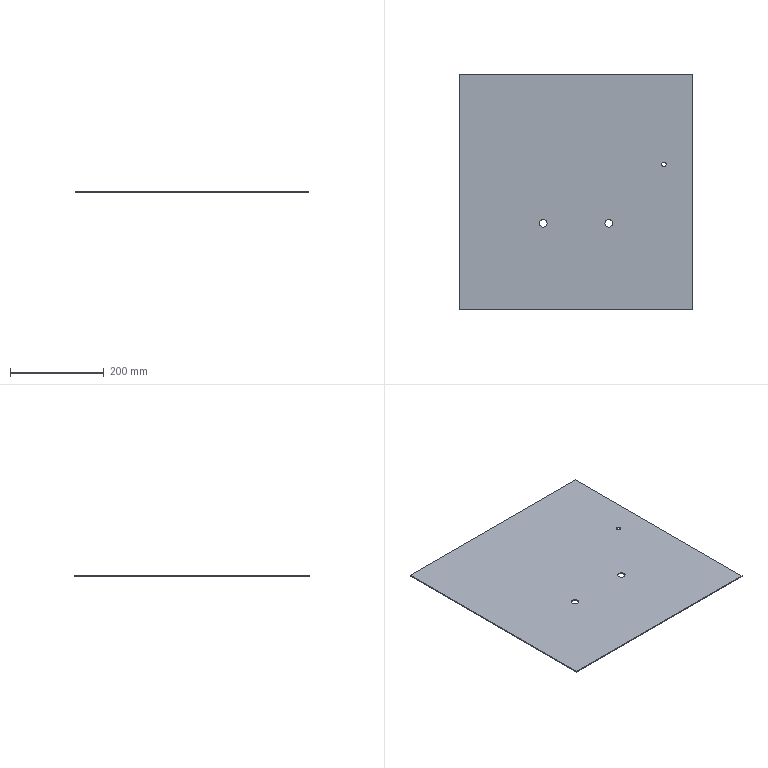Component | SolidWorks | FrameSidePlate2-1 | 1 solid | 12 faces | box 500 x 504 x 2 mm | volume 503039 mm3 | cylinder 6 | plane 6 | commonest cylinder face diameters 16 x4 10 x2
build123d program:
from build123d import *

# Parameters (mm, degrees)
SKETCH1_2_W                   = 500
SKETCH1_2_H                   = 504
BOSS_EXTRUDE1_DEPTH           = 2
SKETCH1_R                     = 8
SKETCH1_R_2                   = 5
REPAIR_SHAFTANDM10HOLES_DEPTH = 10


with BuildPart() as part:
    # Sketch1_2 → Boss-Extrude1 (new body)
    with BuildSketch(Plane.XY):
        Rectangle(SKETCH1_2_W, SKETCH1_2_H)
    extrude(amount=BOSS_EXTRUDE1_DEPTH)

    # Sketch1 → Repair_ShaftAndM10Holes (cut, symmetric)
    with BuildSketch(Plane.XY):
        with Locations((70, -67)):
            Circle(SKETCH1_R)
        with Locations((-70, -67)):
            Circle(SKETCH1_R)
        with Locations((-188, 59)):
            Circle(SKETCH1_R_2)
    extrude(amount=REPAIR_SHAFTANDM10HOLES_DEPTH, both=True, mode=Mode.SUBTRACT)


solid = part.part

# Placed as in the assembly
solid = solid.moved(Location((316.241, -291.715, 1470.724), (-180, 0, 180)))
STEP:
#1=COLOUR_RGB('',0.7922,0.8196,0.9333);
#2=FILL_AREA_STYLE_COLOUR('',#1);
#3=FILL_AREA_STYLE('',(#2));
#4=SURFACE_STYLE_FILL_AREA(#3);
#5=SURFACE_SIDE_STYLE('',(#4));
#6=SURFACE_STYLE_USAGE(.BOTH.,#5);
#7=PRESENTATION_STYLE_ASSIGNMENT((#6));
#8=CARTESIAN_POINT('',(10.009,-14.123,57.903));
#9=VERTEX_POINT('',#8);
#10=CARTESIAN_POINT('',(9.38,-14.123,57.903));
#11=VERTEX_POINT('',#10);
#12=CARTESIAN_POINT('',(9.695,-14.123,57.903));
#13=DIRECTION('',(0.,0.,-1.));
#14=DIRECTION('',(-1.,0.,0.));
#15=AXIS2_PLACEMENT_3D('',#12,#13,#14);
#16=CIRCLE('',#15,0.315);
#17=EDGE_CURVE('',#9,#11,#16,.T.);
#18=ORIENTED_EDGE('',*,*,#17,.F.);
#19=CARTESIAN_POINT('',(10.009,-14.123,57.824));
#20=VERTEX_POINT('',#19);
#21=CARTESIAN_POINT('',(10.009,-14.123,58.296));
#22=DIRECTION('',(0.,0.,-1.));
#23=VECTOR('',#22,39.37);
#24=LINE('',#21,#23);
#25=EDGE_CURVE('',#9,#20,#24,.T.);
#26=ORIENTED_EDGE('',*,*,#25,.T.);
#27=CARTESIAN_POINT('',(9.38,-14.123,57.824));
#28=VERTEX_POINT('',#27);
#29=CARTESIAN_POINT('',(9.695,-14.123,57.824));
#30=DIRECTION('',(0.,0.,-1.));
#31=DIRECTION('',(-1.,0.,0.));
#32=AXIS2_PLACEMENT_3D('',#29,#30,#31);
#33=CIRCLE('',#32,0.315);
#34=EDGE_CURVE('',#20,#28,#33,.T.);
#35=ORIENTED_EDGE('',*,*,#34,.T.);
#36=CARTESIAN_POINT('',(9.38,-14.123,58.296));
#37=DIRECTION('',(0.,0.,-1.));
#38=VECTOR('',#37,39.37);
#39=LINE('',#36,#38);
#40=EDGE_CURVE('',#11,#28,#39,.T.);
#41=ORIENTED_EDGE('',*,*,#40,.F.);
#42=EDGE_LOOP('',(#18,#26,#35,#41));
#43=FACE_OUTER_BOUND('',#42,.T.);
#44=CARTESIAN_POINT('',(9.695,-14.123,58.296));
#45=DIRECTION('',(0.,0.,-1.));
#46=DIRECTION('',(-1.,0.,0.));
#47=AXIS2_PLACEMENT_3D('',#44,#45,#46);
#48=CYLINDRICAL_SURFACE('',#47,0.315);
#49=ADVANCED_FACE('',(#43),#48,.F.);
#50=CARTESIAN_POINT('',(15.521,-14.123,57.903));
#51=VERTEX_POINT('',#50);
#52=CARTESIAN_POINT('',(14.891,-14.123,57.903));
#53=VERTEX_POINT('',#52);
#54=CARTESIAN_POINT('',(15.206,-14.123,57.903));
#55=DIRECTION('',(0.,0.,-1.));
#56=DIRECTION('',(-1.,0.,0.));
#57=AXIS2_PLACEMENT_3D('',#54,#55,#56);
#58=CIRCLE('',#57,0.315);
#59=EDGE_CURVE('',#51,#53,#58,.T.);
#60=ORIENTED_EDGE('',*,*,#59,.F.);
#61=CARTESIAN_POINT('',(15.521,-14.123,57.824));
#62=VERTEX_POINT('',#61);
#63=CARTESIAN_POINT('',(15.521,-14.123,58.296));
#64=DIRECTION('',(0.,0.,-1.));
#65=VECTOR('',#64,39.37);
#66=LINE('',#63,#65);
#67=EDGE_CURVE('',#51,#62,#66,.T.);
#68=ORIENTED_EDGE('',*,*,#67,.T.);
#69=CARTESIAN_POINT('',(14.891,-14.123,57.824));
#70=VERTEX_POINT('',#69);
#71=CARTESIAN_POINT('',(15.206,-14.123,57.824));
#72=DIRECTION('',(0.,0.,-1.));
#73=DIRECTION('',(-1.,0.,0.));
#74=AXIS2_PLACEMENT_3D('',#71,#72,#73);
#75=CIRCLE('',#74,0.315);
#76=EDGE_CURVE('',#62,#70,#75,.T.);
#77=ORIENTED_EDGE('',*,*,#76,.T.);
#78=CARTESIAN_POINT('',(14.891,-14.123,58.296));
#79=DIRECTION('',(0.,0.,-1.));
#80=VECTOR('',#79,39.37);
#81=LINE('',#78,#80);
#82=EDGE_CURVE('',#53,#70,#81,.T.);
#83=ORIENTED_EDGE('',*,*,#82,.F.);
#84=EDGE_LOOP('',(#60,#68,#77,#83));
#85=FACE_OUTER_BOUND('',#84,.T.);
#86=CARTESIAN_POINT('',(15.206,-14.123,58.296));
#87=DIRECTION('',(0.,0.,-1.));
#88=DIRECTION('',(-1.,0.,0.));
#89=AXIS2_PLACEMENT_3D('',#86,#87,#88);
#90=CYLINDRICAL_SURFACE('',#89,0.315);
#91=ADVANCED_FACE('',(#85),#90,.F.);
#92=CARTESIAN_POINT('',(20.049,-9.162,57.903));
#93=VERTEX_POINT('',#92);
#94=CARTESIAN_POINT('',(19.655,-9.162,57.903));
#95=VERTEX_POINT('',#94);
#96=CARTESIAN_POINT('',(19.852,-9.162,57.903));
#97=DIRECTION('',(0.,0.,-1.));
#98=DIRECTION('',(-1.,0.,0.));
#99=AXIS2_PLACEMENT_3D('',#96,#97,#98);
#100=CIRCLE('',#99,0.1969);
#101=EDGE_CURVE('',#93,#95,#100,.T.);
#102=ORIENTED_EDGE('',*,*,#101,.F.);
#103=CARTESIAN_POINT('',(20.049,-9.162,57.824));
#104=VERTEX_POINT('',#103);
#105=CARTESIAN_POINT('',(20.049,-9.162,58.296));
#106=DIRECTION('',(0.,0.,-1.));
#107=VECTOR('',#106,39.37);
#108=LINE('',#105,#107);
#109=EDGE_CURVE('',#93,#104,#108,.T.);
#110=ORIENTED_EDGE('',*,*,#109,.T.);
#111=CARTESIAN_POINT('',(19.655,-9.162,57.824));
#112=VERTEX_POINT('',#111);
#113=CARTESIAN_POINT('',(19.852,-9.162,57.824));
#114=DIRECTION('',(0.,0.,-1.));
#115=DIRECTION('',(-1.,0.,0.));
#116=AXIS2_PLACEMENT_3D('',#113,#114,#115);
#117=CIRCLE('',#116,0.1969);
#118=EDGE_CURVE('',#104,#112,#117,.T.);
#119=ORIENTED_EDGE('',*,*,#118,.T.);
#120=CARTESIAN_POINT('',(19.655,-9.162,58.296));
#121=DIRECTION('',(0.,0.,-1.));
#122=VECTOR('',#121,39.37);
#123=LINE('',#120,#122);
#124=EDGE_CURVE('',#95,#112,#123,.T.);
#125=ORIENTED_EDGE('',*,*,#124,.F.);
#126=EDGE_LOOP('',(#102,#110,#119,#125));
#127=FACE_OUTER_BOUND('',#126,.T.);
#128=CARTESIAN_POINT('',(19.852,-9.162,58.296));
#129=DIRECTION('',(0.,0.,-1.));
#130=DIRECTION('',(-1.,0.,0.));
#131=AXIS2_PLACEMENT_3D('',#128,#129,#130);
#132=CYLINDRICAL_SURFACE('',#131,0.1969);
#133=ADVANCED_FACE('',(#127),#132,.F.);
#134=CARTESIAN_POINT('',(22.293,-1.564,57.903));
#135=VERTEX_POINT('',#134);
#136=CARTESIAN_POINT('',(22.293,-21.406,57.903));
#137=VERTEX_POINT('',#136);
#138=CARTESIAN_POINT('',(22.293,-21.406,57.903));
#139=DIRECTION('',(0.,-1.,0.));
#140=VECTOR('',#139,39.37);
#141=LINE('',#138,#140);
#142=EDGE_CURVE('',#135,#137,#141,.T.);
#143=ORIENTED_EDGE('',*,*,#142,.T.);
#144=CARTESIAN_POINT('',(22.293,-21.406,57.824));
#145=VERTEX_POINT('',#144);
#146=CARTESIAN_POINT('',(22.293,-21.406,57.824));
#147=DIRECTION('',(0.,0.,1.));
#148=VECTOR('',#147,39.37);
#149=LINE('',#146,#148);
#150=EDGE_CURVE('',#145,#137,#149,.T.);
#151=ORIENTED_EDGE('',*,*,#150,.F.);
#152=CARTESIAN_POINT('',(22.293,-1.564,57.824));
#153=VERTEX_POINT('',#152);
#154=CARTESIAN_POINT('',(22.293,-21.406,57.824));
#155=DIRECTION('',(0.,-1.,0.));
#156=VECTOR('',#155,39.37);
#157=LINE('',#154,#156);
#158=EDGE_CURVE('',#153,#145,#157,.T.);
#159=ORIENTED_EDGE('',*,*,#158,.F.);
#160=CARTESIAN_POINT('',(22.293,-1.564,57.824));
#161=DIRECTION('',(0.,0.,1.));
#162=VECTOR('',#161,39.37);
#163=LINE('',#160,#162);
#164=EDGE_CURVE('',#153,#135,#163,.T.);
#165=ORIENTED_EDGE('',*,*,#164,.T.);
#166=EDGE_LOOP('',(#143,#151,#159,#165));
#167=FACE_OUTER_BOUND('',#166,.T.);
#168=CARTESIAN_POINT('',(22.293,-21.406,57.824));
#169=DIRECTION('',(-1.,0.,0.));
#170=DIRECTION('',(0.,0.,1.));
#171=AXIS2_PLACEMENT_3D('',#168,#169,#170);
#172=PLANE('',#171);
#173=ADVANCED_FACE('',(#167),#172,.F.);
#174=CARTESIAN_POINT('',(2.608,-21.406,57.903));
#175=VERTEX_POINT('',#174);
#176=CARTESIAN_POINT('',(2.608,-21.406,57.903));
#177=DIRECTION('',(-1.,0.,0.));
#178=VECTOR('',#177,39.37);
#179=LINE('',#176,#178);
#180=EDGE_CURVE('',#137,#175,#179,.T.);
#181=ORIENTED_EDGE('',*,*,#180,.T.);
#182=CARTESIAN_POINT('',(2.608,-21.406,57.824));
#183=VERTEX_POINT('',#182);
#184=CARTESIAN_POINT('',(2.608,-21.406,57.824));
#185=DIRECTION('',(0.,0.,1.));
#186=VECTOR('',#185,39.37);
#187=LINE('',#184,#186);
#188=EDGE_CURVE('',#183,#175,#187,.T.);
#189=ORIENTED_EDGE('',*,*,#188,.F.);
#190=CARTESIAN_POINT('',(2.608,-21.406,57.824));
#191=DIRECTION('',(-1.,0.,0.));
#192=VECTOR('',#191,39.37);
#193=LINE('',#190,#192);
#194=EDGE_CURVE('',#145,#183,#193,.T.);
#195=ORIENTED_EDGE('',*,*,#194,.F.);
#196=ORIENTED_EDGE('',*,*,#150,.T.);
#197=EDGE_LOOP('',(#181,#189,#195,#196));
#198=FACE_OUTER_BOUND('',#197,.T.);
#199=CARTESIAN_POINT('',(2.608,-21.406,57.824));
#200=DIRECTION('',(0.,1.,0.));
#201=DIRECTION('',(0.,0.,-1.));
#202=AXIS2_PLACEMENT_3D('',#199,#200,#201);
#203=PLANE('',#202);
#204=ADVANCED_FACE('',(#198),#203,.F.);
#205=CARTESIAN_POINT('',(2.608,-1.564,57.903));
#206=VERTEX_POINT('',#205);
#207=CARTESIAN_POINT('',(2.608,-21.406,57.903));
#208=DIRECTION('',(0.,1.,0.));
#209=VECTOR('',#208,39.37);
#210=LINE('',#207,#209);
#211=EDGE_CURVE('',#175,#206,#210,.T.);
#212=ORIENTED_EDGE('',*,*,#211,.T.);
#213=CARTESIAN_POINT('',(2.608,-1.564,57.824));
#214=VERTEX_POINT('',#213);
#215=CARTESIAN_POINT('',(2.608,-1.564,57.824));
#216=DIRECTION('',(0.,0.,1.));
#217=VECTOR('',#216,39.37);
#218=LINE('',#215,#217);
#219=EDGE_CURVE('',#214,#206,#218,.T.);
#220=ORIENTED_EDGE('',*,*,#219,.F.);
#221=CARTESIAN_POINT('',(2.608,-21.406,57.824));
#222=DIRECTION('',(0.,1.,0.));
#223=VECTOR('',#222,39.37);
#224=LINE('',#221,#223);
#225=EDGE_CURVE('',#183,#214,#224,.T.);
#226=ORIENTED_EDGE('',*,*,#225,.F.);
#227=ORIENTED_EDGE('',*,*,#188,.T.);
#228=EDGE_LOOP('',(#212,#220,#226,#227));
#229=FACE_OUTER_BOUND('',#228,.T.);
#230=CARTESIAN_POINT('',(2.608,-21.406,57.824));
#231=DIRECTION('',(1.,0.,0.));
#232=DIRECTION('',(0.,0.,-1.));
#233=AXIS2_PLACEMENT_3D('',#230,#231,#232);
#234=PLANE('',#233);
#235=ADVANCED_FACE('',(#229),#234,.F.);
#236=CARTESIAN_POINT('',(2.608,-1.564,57.903));
#237=DIRECTION('',(1.,-0.,0.));
#238=VECTOR('',#237,39.37);
#239=LINE('',#236,#238);
#240=EDGE_CURVE('',#206,#135,#239,.T.);
#241=ORIENTED_EDGE('',*,*,#240,.T.);
#242=ORIENTED_EDGE('',*,*,#164,.F.);
#243=CARTESIAN_POINT('',(2.608,-1.564,57.824));
#244=DIRECTION('',(1.,-0.,0.));
#245=VECTOR('',#244,39.37);
#246=LINE('',#243,#245);
#247=EDGE_CURVE('',#214,#153,#246,.T.);
#248=ORIENTED_EDGE('',*,*,#247,.F.);
#249=ORIENTED_EDGE('',*,*,#219,.T.);
#250=EDGE_LOOP('',(#241,#242,#248,#249));
#251=FACE_OUTER_BOUND('',#250,.T.);
#252=CARTESIAN_POINT('',(2.608,-1.564,57.824));
#253=DIRECTION('',(-0.,-1.,0.));
#254=DIRECTION('',(-1.,0.,0.));
#255=AXIS2_PLACEMENT_3D('',#252,#253,#254);
#256=PLANE('',#255);
#257=ADVANCED_FACE('',(#251),#256,.F.);
#258=CARTESIAN_POINT('',(9.695,-14.123,57.824));
#259=DIRECTION('',(0.,0.,-1.));
#260=DIRECTION('',(-1.,0.,0.));
#261=AXIS2_PLACEMENT_3D('',#258,#259,#260);
#262=CIRCLE('',#261,0.315);
#263=EDGE_CURVE('',#28,#20,#262,.T.);
#264=ORIENTED_EDGE('',*,*,#263,.F.);
#265=ORIENTED_EDGE('',*,*,#34,.F.);
#266=EDGE_LOOP('',(#264,#265));
#267=FACE_BOUND('',#266,.T.);
#268=CARTESIAN_POINT('',(15.206,-14.123,57.824));
#269=DIRECTION('',(0.,0.,-1.));
#270=DIRECTION('',(-1.,0.,0.));
#271=AXIS2_PLACEMENT_3D('',#268,#269,#270);
#272=CIRCLE('',#271,0.315);
#273=EDGE_CURVE('',#70,#62,#272,.T.);
#274=ORIENTED_EDGE('',*,*,#273,.F.);
#275=ORIENTED_EDGE('',*,*,#76,.F.);
#276=EDGE_LOOP('',(#274,#275));
#277=FACE_BOUND('',#276,.T.);
#278=CARTESIAN_POINT('',(19.852,-9.162,57.824));
#279=DIRECTION('',(0.,0.,-1.));
#280=DIRECTION('',(-1.,0.,0.));
#281=AXIS2_PLACEMENT_3D('',#278,#279,#280);
#282=CIRCLE('',#281,0.1969);
#283=EDGE_CURVE('',#112,#104,#282,.T.);
#284=ORIENTED_EDGE('',*,*,#283,.F.);
#285=ORIENTED_EDGE('',*,*,#118,.F.);
#286=EDGE_LOOP('',(#284,#285));
#287=FACE_BOUND('',#286,.T.);
#288=ORIENTED_EDGE('',*,*,#158,.T.);
#289=ORIENTED_EDGE('',*,*,#194,.T.);
#290=ORIENTED_EDGE('',*,*,#225,.T.);
#291=ORIENTED_EDGE('',*,*,#247,.T.);
#292=EDGE_LOOP('',(#288,#289,#290,#291));
#293=FACE_OUTER_BOUND('',#292,.T.);
#294=CARTESIAN_POINT('',(12.45,-11.485,57.824));
#295=DIRECTION('',(0.,0.,-1.));
#296=DIRECTION('',(-1.,0.,0.));
#297=AXIS2_PLACEMENT_3D('',#294,#295,#296);
#298=PLANE('',#297);
#299=ADVANCED_FACE('',(#267,#277,#287,#293),#298,.T.);
#300=CARTESIAN_POINT('',(9.695,-14.123,57.903));
#301=DIRECTION('',(0.,0.,-1.));
#302=DIRECTION('',(-1.,0.,0.));
#303=AXIS2_PLACEMENT_3D('',#300,#301,#302);
#304=CIRCLE('',#303,0.315);
#305=EDGE_CURVE('',#11,#9,#304,.T.);
#306=ORIENTED_EDGE('',*,*,#305,.T.);
#307=ORIENTED_EDGE('',*,*,#17,.T.);
#308=EDGE_LOOP('',(#306,#307));
#309=FACE_BOUND('',#308,.T.);
#310=CARTESIAN_POINT('',(15.206,-14.123,57.903));
#311=DIRECTION('',(0.,0.,-1.));
#312=DIRECTION('',(-1.,0.,0.));
#313=AXIS2_PLACEMENT_3D('',#310,#311,#312);
#314=CIRCLE('',#313,0.315);
#315=EDGE_CURVE('',#53,#51,#314,.T.);
#316=ORIENTED_EDGE('',*,*,#315,.T.);
#317=ORIENTED_EDGE('',*,*,#59,.T.);
#318=EDGE_LOOP('',(#316,#317));
#319=FACE_BOUND('',#318,.T.);
#320=CARTESIAN_POINT('',(19.852,-9.162,57.903));
#321=DIRECTION('',(0.,0.,-1.));
#322=DIRECTION('',(-1.,0.,0.));
#323=AXIS2_PLACEMENT_3D('',#320,#321,#322);
#324=CIRCLE('',#323,0.1969);
#325=EDGE_CURVE('',#95,#93,#324,.T.);
#326=ORIENTED_EDGE('',*,*,#325,.T.);
#327=ORIENTED_EDGE('',*,*,#101,.T.);
#328=EDGE_LOOP('',(#326,#327));
#329=FACE_BOUND('',#328,.T.);
#330=ORIENTED_EDGE('',*,*,#142,.F.);
#331=ORIENTED_EDGE('',*,*,#240,.F.);
#332=ORIENTED_EDGE('',*,*,#211,.F.);
#333=ORIENTED_EDGE('',*,*,#180,.F.);
#334=EDGE_LOOP('',(#330,#331,#332,#333));
#335=FACE_OUTER_BOUND('',#334,.T.);
#336=CARTESIAN_POINT('',(12.45,-11.485,57.903));
#337=DIRECTION('',(0.,0.,-1.));
#338=DIRECTION('',(-1.,0.,0.));
#339=AXIS2_PLACEMENT_3D('',#336,#337,#338);
#340=PLANE('',#339);
#341=ADVANCED_FACE('',(#309,#319,#329,#335),#340,.F.);
#342=ORIENTED_EDGE('',*,*,#109,.F.);
#343=ORIENTED_EDGE('',*,*,#325,.F.);
#344=ORIENTED_EDGE('',*,*,#124,.T.);
#345=ORIENTED_EDGE('',*,*,#283,.T.);
#346=EDGE_LOOP('',(#342,#343,#344,#345));
#347=FACE_OUTER_BOUND('',#346,.T.);
#348=CARTESIAN_POINT('',(19.852,-9.162,58.296));
#349=DIRECTION('',(0.,0.,-1.));
#350=DIRECTION('',(-1.,0.,0.));
#351=AXIS2_PLACEMENT_3D('',#348,#349,#350);
#352=CYLINDRICAL_SURFACE('',#351,0.1969);
#353=ADVANCED_FACE('',(#347),#352,.F.);
#354=ORIENTED_EDGE('',*,*,#67,.F.);
#355=ORIENTED_EDGE('',*,*,#315,.F.);
#356=ORIENTED_EDGE('',*,*,#82,.T.);
#357=ORIENTED_EDGE('',*,*,#273,.T.);
#358=EDGE_LOOP('',(#354,#355,#356,#357));
#359=FACE_OUTER_BOUND('',#358,.T.);
#360=CARTESIAN_POINT('',(15.206,-14.123,58.296));
#361=DIRECTION('',(0.,0.,-1.));
#362=DIRECTION('',(-1.,0.,0.));
#363=AXIS2_PLACEMENT_3D('',#360,#361,#362);
#364=CYLINDRICAL_SURFACE('',#363,0.315);
#365=ADVANCED_FACE('',(#359),#364,.F.);
#366=ORIENTED_EDGE('',*,*,#25,.F.);
#367=ORIENTED_EDGE('',*,*,#305,.F.);
#368=ORIENTED_EDGE('',*,*,#40,.T.);
#369=ORIENTED_EDGE('',*,*,#263,.T.);
#370=EDGE_LOOP('',(#366,#367,#368,#369));
#371=FACE_OUTER_BOUND('',#370,.T.);
#372=CARTESIAN_POINT('',(9.695,-14.123,58.296));
#373=DIRECTION('',(0.,0.,-1.));
#374=DIRECTION('',(-1.,0.,0.));
#375=AXIS2_PLACEMENT_3D('',#372,#373,#374);
#376=CYLINDRICAL_SURFACE('',#375,0.315);
#377=ADVANCED_FACE('',(#371),#376,.F.);
#378=CLOSED_SHELL('',(#49,#91,#133,#173,#204,#235,#257,#299,#341,#353,#365,#377));
#379=MANIFOLD_SOLID_BREP('',#378);
#380=STYLED_ITEM('',(#7),#379);
#381=PRESENTATION_LAYER_ASSIGNMENT('','',(#380));
#382=(LENGTH_UNIT()NAMED_UNIT(*)SI_UNIT($,.METRE.));
#383=LENGTH_MEASURE_WITH_UNIT(LENGTH_MEASURE(0.0254),#382);
#384=DIMENSIONAL_EXPONENTS(1.,0.,0.,0.,0.,0.,0.);
#385=(CONVERSION_BASED_UNIT('',#383)LENGTH_UNIT()NAMED_UNIT(#384));
#386=UNCERTAINTY_MEASURE_WITH_UNIT(LENGTH_MEASURE(0.00001),#385,'','');
#387=(NAMED_UNIT(*)PLANE_ANGLE_UNIT()SI_UNIT($,.RADIAN.));
#388=(NAMED_UNIT(*)SI_UNIT($,.STERADIAN.)SOLID_ANGLE_UNIT());
#389=(GEOMETRIC_REPRESENTATION_CONTEXT(3)GLOBAL_UNCERTAINTY_ASSIGNED_CONTEXT((#386))GLOBAL_UNIT_ASSIGNED_CONTEXT((#385,#387,#388))REPRESENTATION_CONTEXT('',''));
#390=MECHANICAL_DESIGN_GEOMETRIC_PRESENTATION_REPRESENTATION('',(#380),#389);
#391=CARTESIAN_POINT('',(0.,0.,0.));
#392=DIRECTION('',(0.,0.,1.));
#393=DIRECTION('',(1.,0.,0.));
#394=AXIS2_PLACEMENT_3D('',#391,#392,#393);
#395=(LENGTH_UNIT()NAMED_UNIT(*)SI_UNIT($,.METRE.));
#396=LENGTH_MEASURE_WITH_UNIT(LENGTH_MEASURE(0.0254),#395);
#397=DIMENSIONAL_EXPONENTS(1.,0.,0.,0.,0.,0.,0.);
#398=(CONVERSION_BASED_UNIT('',#396)LENGTH_UNIT()NAMED_UNIT(#397));
#399=UNCERTAINTY_MEASURE_WITH_UNIT(LENGTH_MEASURE(0.00001),#398,'','');
#400=(NAMED_UNIT(*)PLANE_ANGLE_UNIT()SI_UNIT($,.RADIAN.));
#401=(NAMED_UNIT(*)SI_UNIT($,.STERADIAN.)SOLID_ANGLE_UNIT());
#402=(GEOMETRIC_REPRESENTATION_CONTEXT(3)GLOBAL_UNCERTAINTY_ASSIGNED_CONTEXT((#399))GLOBAL_UNIT_ASSIGNED_CONTEXT((#398,#400,#401))REPRESENTATION_CONTEXT('',''));
#403=ADVANCED_BREP_SHAPE_REPRESENTATION('',(#379,#394),#402);